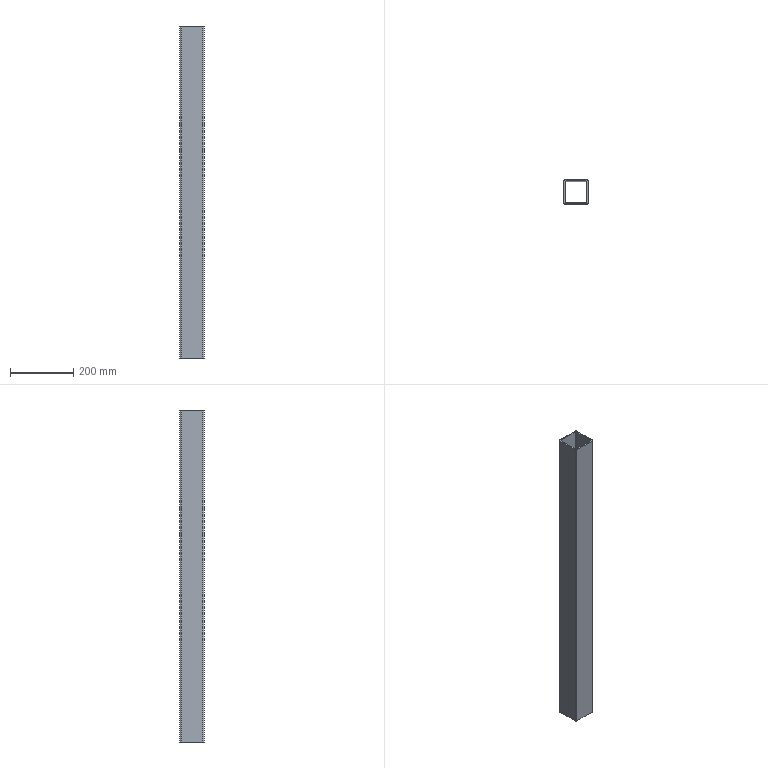Component | NX | BASE_FRAME_SQ_TUBE | 1 solid | 18 faces | volume 1212960 mm3 | plane 10 | cylinder 8 | commonest cylinder face diameters 8 x8